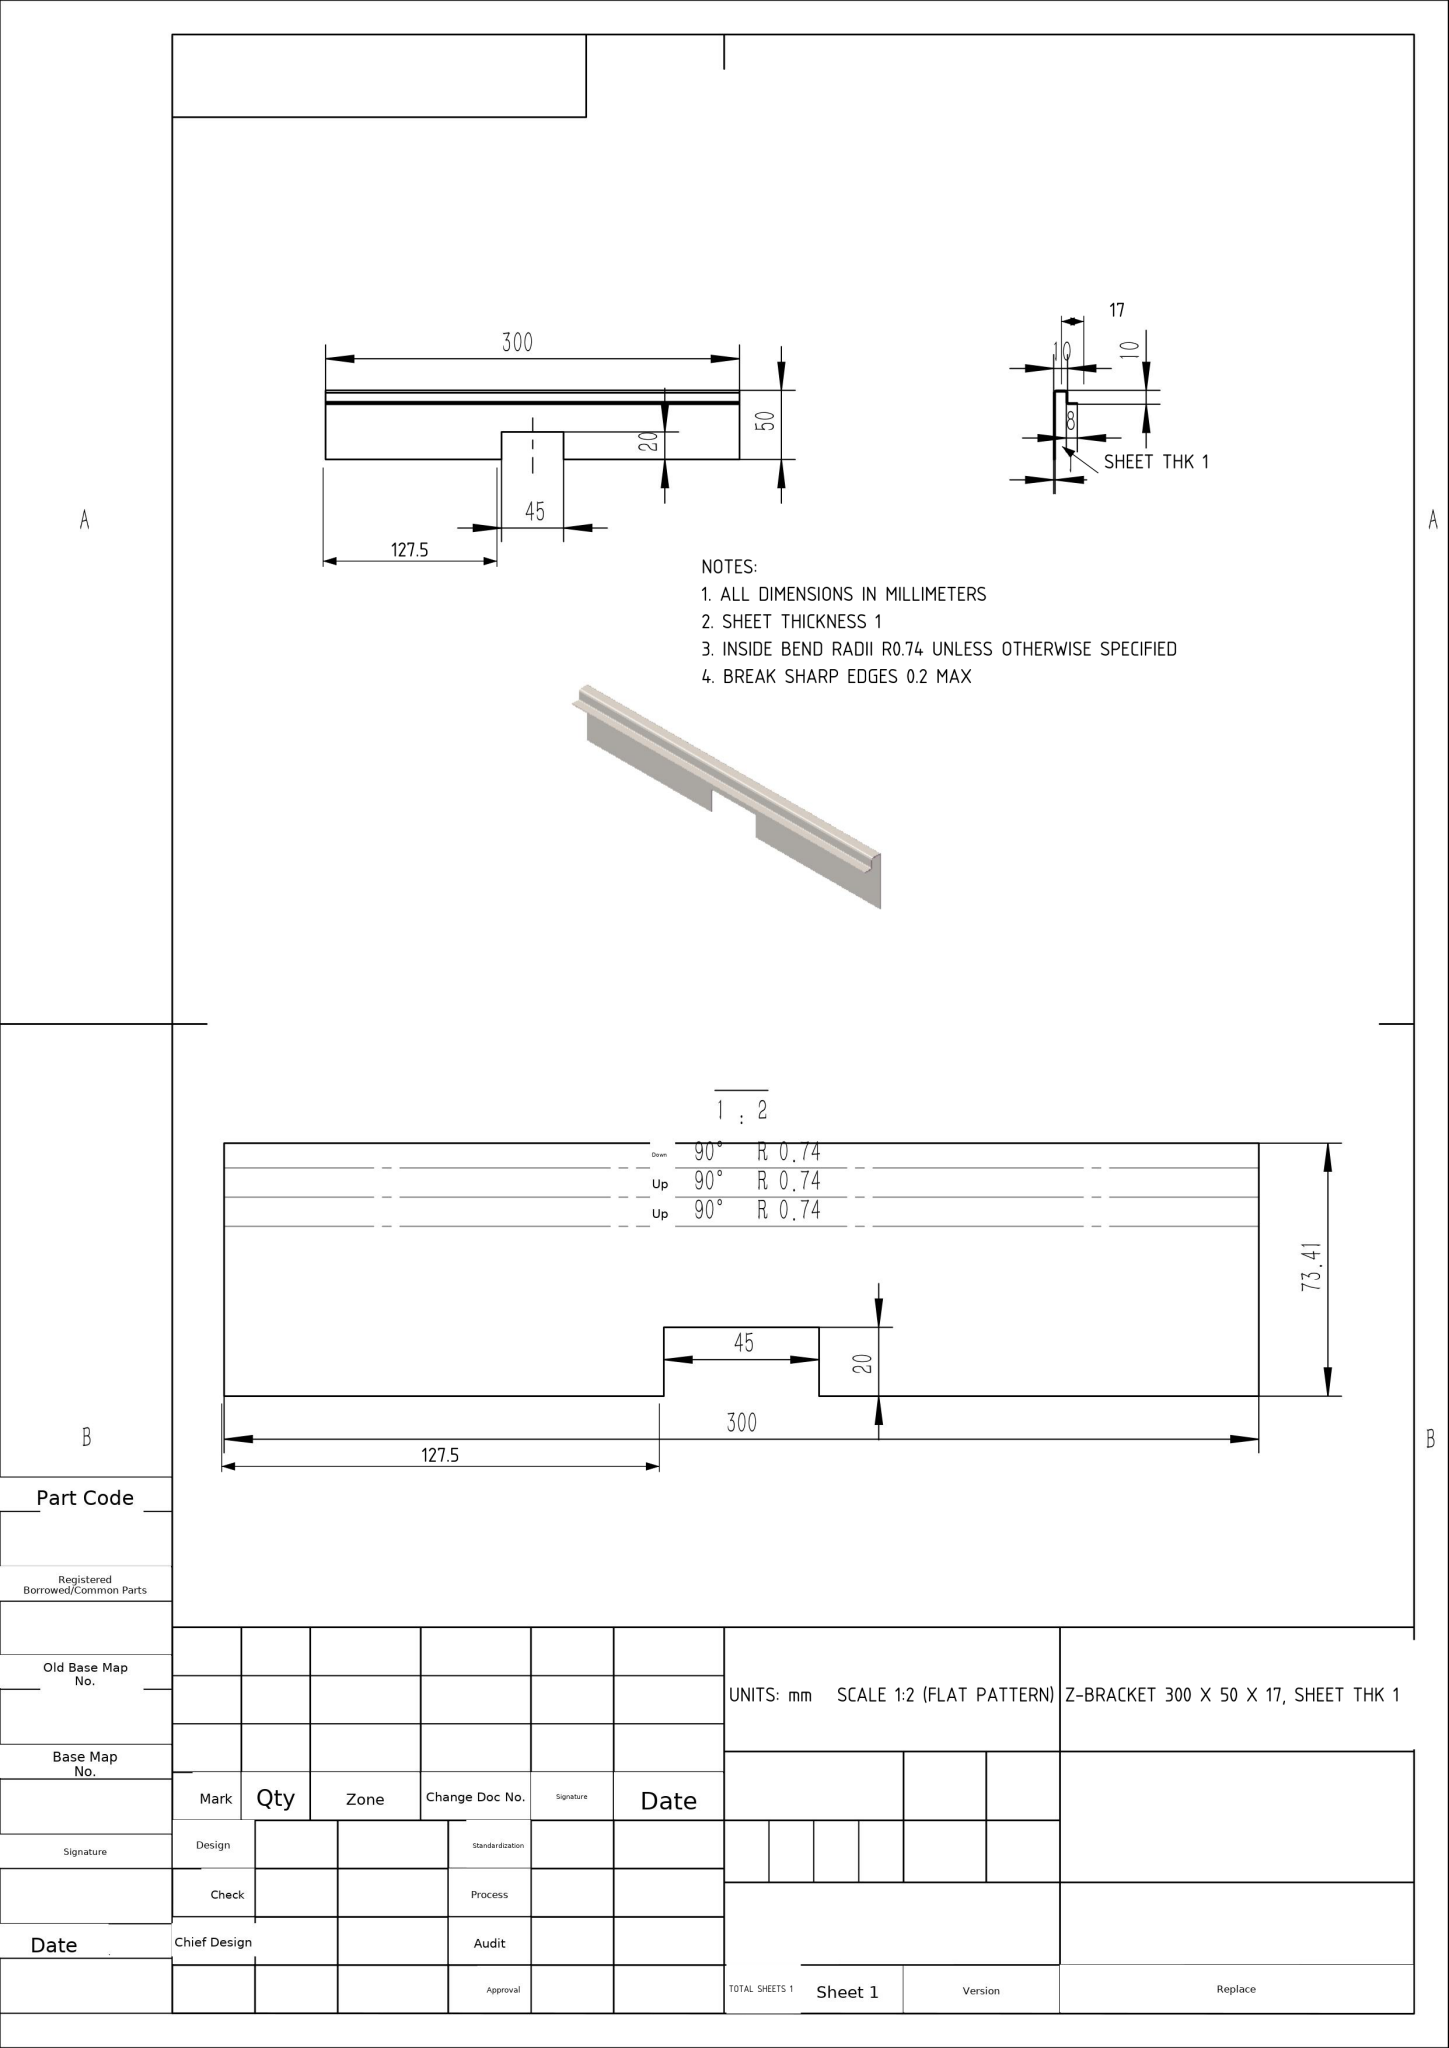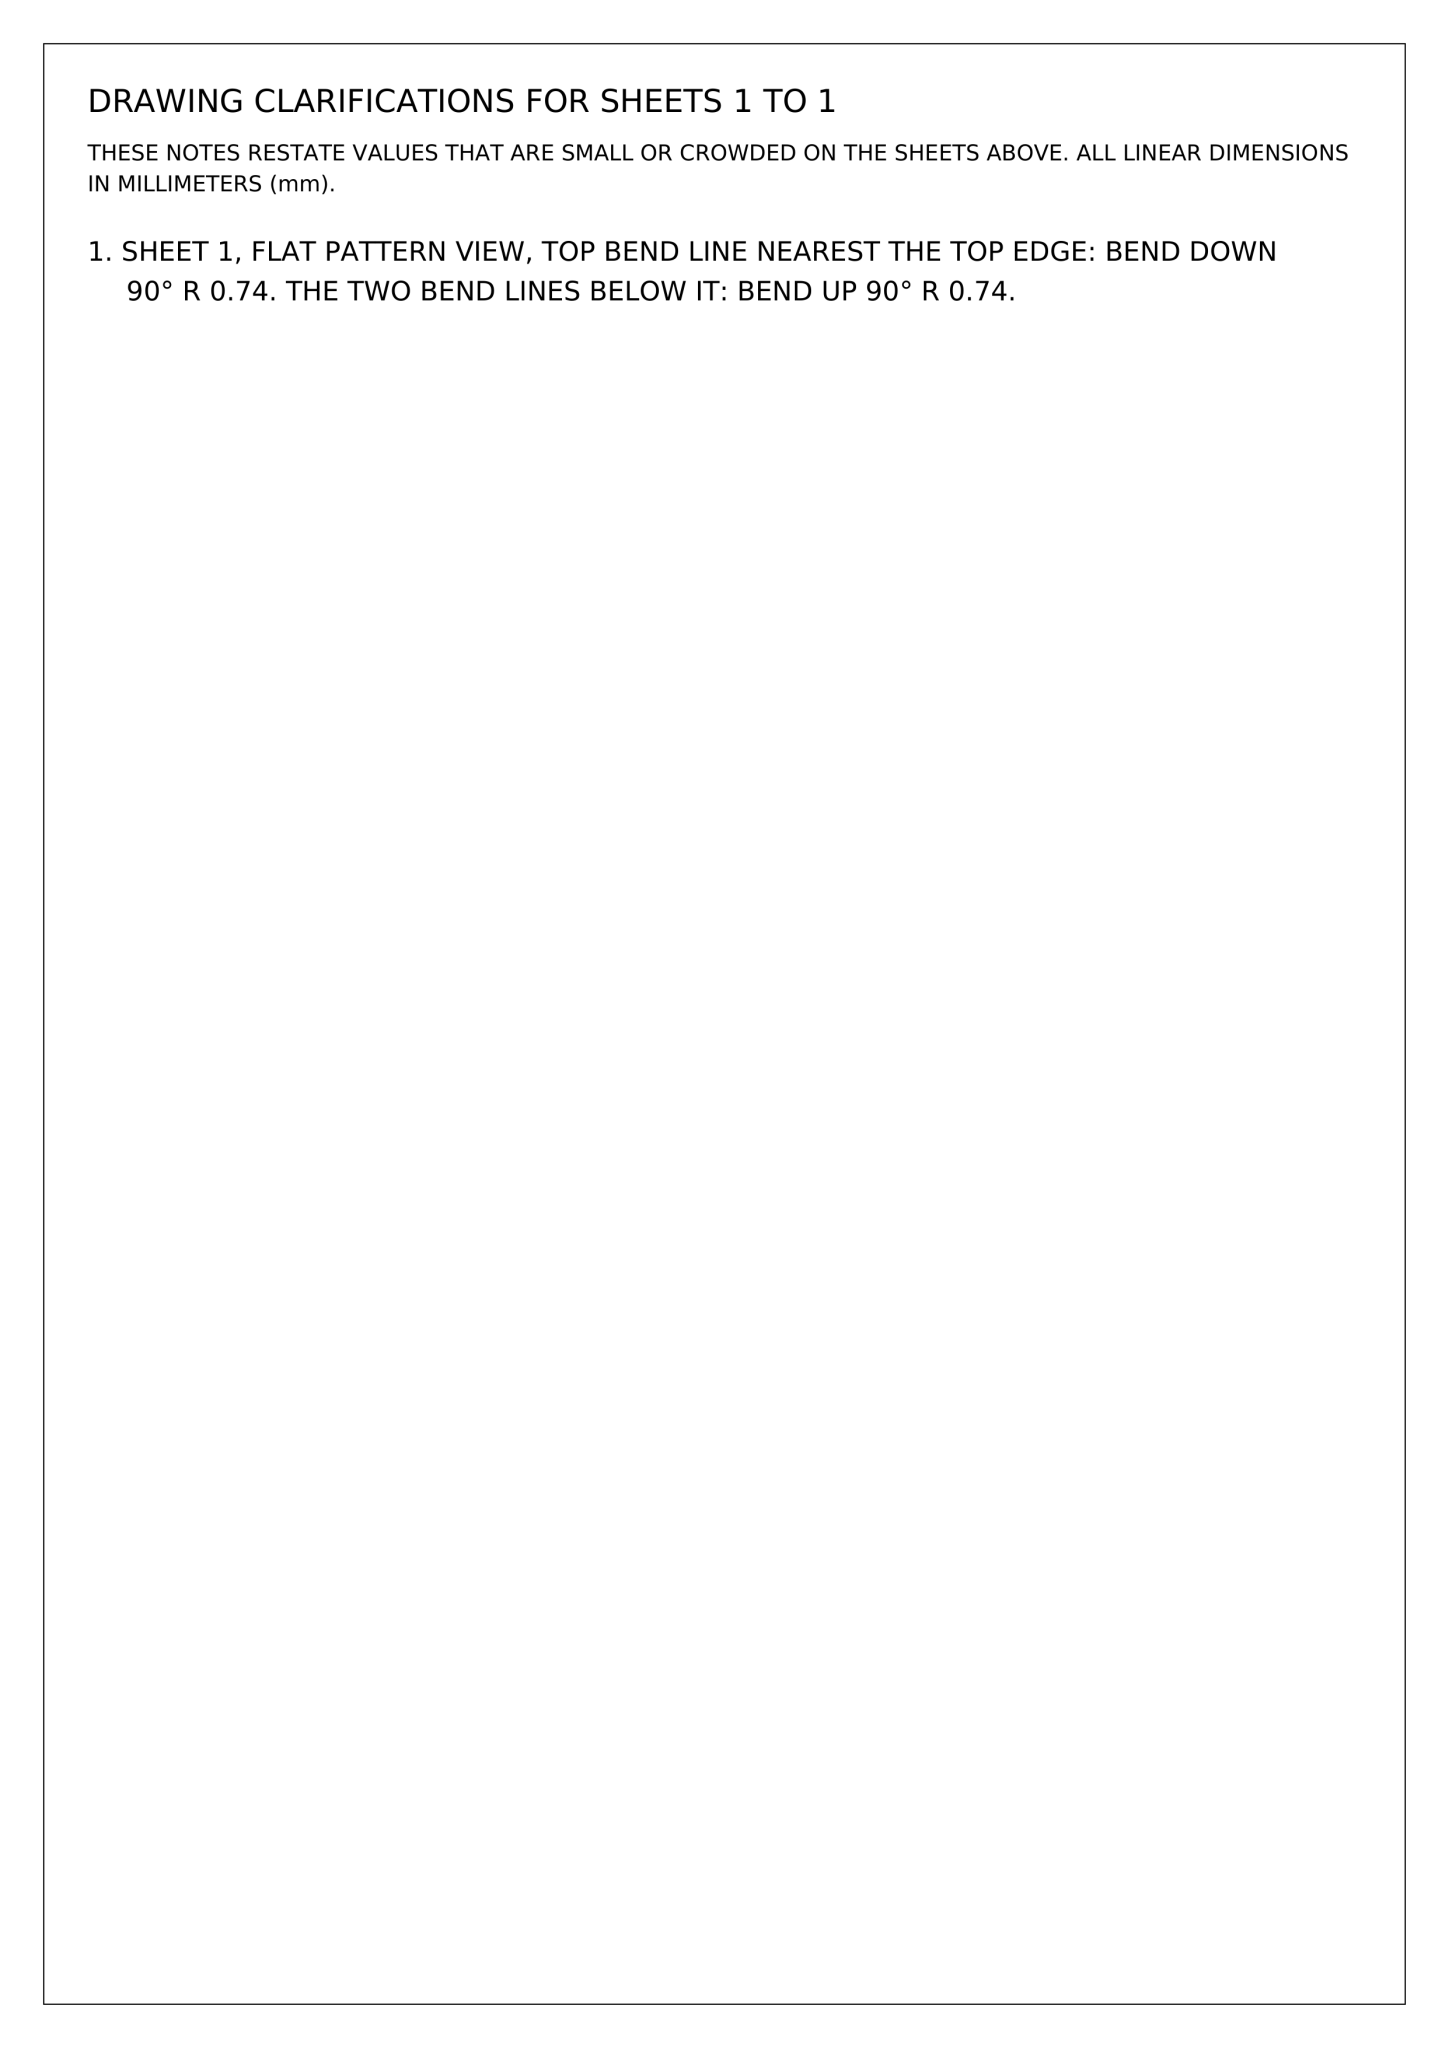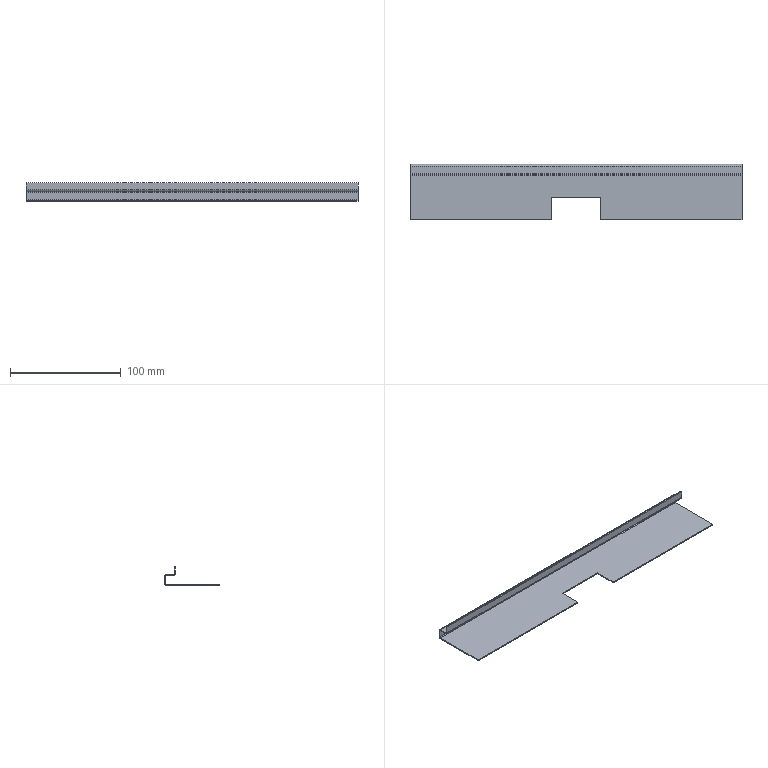Part | NX | mm | 1 solid | 34 faces | box 300 x 50 x 17 mm | volume 21122 mm3 | plane 28 | cylinder 6 | commonest cylinder face diameters 3.473 x3 1.473 x3
STEP:
#1=COLOUR_RGB('',0.6471,0.6196,0.5882);
#2=FILL_AREA_STYLE_COLOUR('',#1);
#3=FILL_AREA_STYLE('',(#2));
#4=SURFACE_STYLE_FILL_AREA(#3);
#5=SURFACE_SIDE_STYLE('',(#4));
#6=SURFACE_STYLE_USAGE(.BOTH.,#5);
#7=PRESENTATION_STYLE_ASSIGNMENT((#6));
#8=CARTESIAN_POINT('',(13.846,64.904,-1.));
#9=VERTEX_POINT('',#8);
#10=CARTESIAN_POINT('',(13.846,64.904,0.));
#11=VERTEX_POINT('',#10);
#12=CARTESIAN_POINT('',(13.846,64.904,-1.));
#13=DIRECTION('',(0.,0.,1.));
#14=VECTOR('',#13,1000.);
#15=LINE('',#12,#14);
#16=EDGE_CURVE('',#9,#11,#15,.T.);
#17=ORIENTED_EDGE('',*,*,#16,.F.);
#18=CARTESIAN_POINT('',(141.346,64.904,-1.));
#19=VERTEX_POINT('',#18);
#20=CARTESIAN_POINT('',(-158.654,64.904,-1.));
#21=DIRECTION('',(1.,0.,0.));
#22=VECTOR('',#21,1000.);
#23=LINE('',#20,#22);
#24=EDGE_CURVE('',#9,#19,#23,.T.);
#25=ORIENTED_EDGE('',*,*,#24,.T.);
#26=CARTESIAN_POINT('',(141.346,64.904,0.));
#27=VERTEX_POINT('',#26);
#28=CARTESIAN_POINT('',(141.346,64.904,-1.));
#29=DIRECTION('',(0.,0.,1.));
#30=VECTOR('',#29,1000.);
#31=LINE('',#28,#30);
#32=EDGE_CURVE('',#19,#27,#31,.T.);
#33=ORIENTED_EDGE('',*,*,#32,.T.);
#34=CARTESIAN_POINT('',(-158.654,64.904,0.));
#35=DIRECTION('',(1.,0.,0.));
#36=VECTOR('',#35,1000.);
#37=LINE('',#34,#36);
#38=EDGE_CURVE('',#11,#27,#37,.T.);
#39=ORIENTED_EDGE('',*,*,#38,.F.);
#40=EDGE_LOOP('',(#17,#25,#33,#39));
#41=FACE_OUTER_BOUND('',#40,.T.);
#42=CARTESIAN_POINT('',(-158.654,64.904,-1.));
#43=DIRECTION('',(0.,-1.,0.));
#44=DIRECTION('',(0.,0.,-1.));
#45=AXIS2_PLACEMENT_3D('',#42,#43,#44);
#46=PLANE('',#45);
#47=ADVANCED_FACE('',(#41),#46,.T.);
#48=CARTESIAN_POINT('',(141.346,113.167,9.));
#49=VERTEX_POINT('',#48);
#50=CARTESIAN_POINT('',(141.346,106.64,9.));
#51=VERTEX_POINT('',#50);
#52=CARTESIAN_POINT('',(141.346,104.904,9.));
#53=DIRECTION('',(0.,-1.,0.));
#54=VECTOR('',#53,1000.);
#55=LINE('',#52,#54);
#56=EDGE_CURVE('',#49,#51,#55,.T.);
#57=ORIENTED_EDGE('',*,*,#56,.T.);
#58=CARTESIAN_POINT('',(141.346,106.64,8.));
#59=VERTEX_POINT('',#58);
#60=CARTESIAN_POINT('',(141.346,106.64,9.));
#61=DIRECTION('',(0.,0.,-1.));
#62=VECTOR('',#61,1000.);
#63=LINE('',#60,#62);
#64=EDGE_CURVE('',#51,#59,#63,.T.);
#65=ORIENTED_EDGE('',*,*,#64,.T.);
#66=CARTESIAN_POINT('',(141.346,113.167,8.));
#67=VERTEX_POINT('',#66);
#68=CARTESIAN_POINT('',(141.346,0.,8.));
#69=DIRECTION('',(0.,-1.,0.));
#70=VECTOR('',#69,1000.);
#71=LINE('',#68,#70);
#72=EDGE_CURVE('',#67,#59,#71,.T.);
#73=ORIENTED_EDGE('',*,*,#72,.F.);
#74=CARTESIAN_POINT('',(141.346,113.167,9.));
#75=DIRECTION('',(0.,0.,1.));
#76=VECTOR('',#75,1000.);
#77=LINE('',#74,#76);
#78=EDGE_CURVE('',#67,#49,#77,.T.);
#79=ORIENTED_EDGE('',*,*,#78,.T.);
#80=EDGE_LOOP('',(#57,#65,#73,#79));
#81=FACE_OUTER_BOUND('',#80,.T.);
#82=CARTESIAN_POINT('',(141.346,104.904,9.));
#83=DIRECTION('',(1.,0.,0.));
#84=DIRECTION('',(0.,0.,-1.));
#85=AXIS2_PLACEMENT_3D('',#82,#83,#84);
#86=PLANE('',#85);
#87=ADVANCED_FACE('',(#81),#86,.T.);
#88=CARTESIAN_POINT('',(-158.654,106.64,9.));
#89=VERTEX_POINT('',#88);
#90=CARTESIAN_POINT('',(-158.654,113.167,9.));
#91=VERTEX_POINT('',#90);
#92=CARTESIAN_POINT('',(-158.654,113.904,9.));
#93=DIRECTION('',(0.,1.,-0.));
#94=VECTOR('',#93,1000.);
#95=LINE('',#92,#94);
#96=EDGE_CURVE('',#89,#91,#95,.T.);
#97=ORIENTED_EDGE('',*,*,#96,.F.);
#98=CARTESIAN_POINT('',(141.346,106.64,9.));
#99=DIRECTION('',(-1.,0.,0.));
#100=VECTOR('',#99,1000.);
#101=LINE('',#98,#100);
#102=EDGE_CURVE('',#51,#89,#101,.T.);
#103=ORIENTED_EDGE('',*,*,#102,.F.);
#104=ORIENTED_EDGE('',*,*,#56,.F.);
#105=CARTESIAN_POINT('',(0.,113.167,9.));
#106=DIRECTION('',(-1.,0.,0.));
#107=VECTOR('',#106,1000.);
#108=LINE('',#105,#107);
#109=EDGE_CURVE('',#49,#91,#108,.T.);
#110=ORIENTED_EDGE('',*,*,#109,.T.);
#111=EDGE_LOOP('',(#97,#103,#104,#110));
#112=FACE_OUTER_BOUND('',#111,.T.);
#113=CARTESIAN_POINT('',(0.,0.,9.));
#114=DIRECTION('',(0.,0.,1.));
#115=DIRECTION('',(0.,-1.,0.));
#116=AXIS2_PLACEMENT_3D('',#113,#114,#115);
#117=PLANE('',#116);
#118=ADVANCED_FACE('',(#112),#117,.T.);
#119=CARTESIAN_POINT('',(-158.654,106.64,8.));
#120=VERTEX_POINT('',#119);
#121=CARTESIAN_POINT('',(141.346,106.64,8.));
#122=DIRECTION('',(-1.,0.,0.));
#123=VECTOR('',#122,1000.);
#124=LINE('',#121,#123);
#125=EDGE_CURVE('',#59,#120,#124,.T.);
#126=ORIENTED_EDGE('',*,*,#125,.T.);
#127=CARTESIAN_POINT('',(-158.654,113.167,8.));
#128=VERTEX_POINT('',#127);
#129=CARTESIAN_POINT('',(-158.654,0.,8.));
#130=DIRECTION('',(0.,1.,-0.));
#131=VECTOR('',#130,1000.);
#132=LINE('',#129,#131);
#133=EDGE_CURVE('',#120,#128,#132,.T.);
#134=ORIENTED_EDGE('',*,*,#133,.T.);
#135=CARTESIAN_POINT('',(141.346,113.167,8.));
#136=DIRECTION('',(-1.,0.,0.));
#137=VECTOR('',#136,1000.);
#138=LINE('',#135,#137);
#139=EDGE_CURVE('',#67,#128,#138,.T.);
#140=ORIENTED_EDGE('',*,*,#139,.F.);
#141=ORIENTED_EDGE('',*,*,#72,.T.);
#142=EDGE_LOOP('',(#126,#134,#140,#141));
#143=FACE_OUTER_BOUND('',#142,.T.);
#144=CARTESIAN_POINT('',(0.,0.,8.));
#145=DIRECTION('',(0.,0.,1.));
#146=DIRECTION('',(0.,-1.,0.));
#147=AXIS2_PLACEMENT_3D('',#144,#145,#146);
#148=PLANE('',#147);
#149=ADVANCED_FACE('',(#143),#148,.F.);
#150=CARTESIAN_POINT('',(141.346,113.904,7.263));
#151=VERTEX_POINT('',#150);
#152=CARTESIAN_POINT('',(141.346,114.904,7.263));
#153=VERTEX_POINT('',#152);
#154=CARTESIAN_POINT('',(141.346,113.904,7.263));
#155=DIRECTION('',(0.,1.,-0.));
#156=VECTOR('',#155,1000.);
#157=LINE('',#154,#156);
#158=EDGE_CURVE('',#151,#153,#157,.T.);
#159=ORIENTED_EDGE('',*,*,#158,.F.);
#160=CARTESIAN_POINT('',(141.346,113.904,0.7366));
#161=VERTEX_POINT('',#160);
#162=CARTESIAN_POINT('',(141.346,113.904,-0.));
#163=DIRECTION('',(0.,-0.,-1.));
#164=VECTOR('',#163,1000.);
#165=LINE('',#162,#164);
#166=EDGE_CURVE('',#151,#161,#165,.T.);
#167=ORIENTED_EDGE('',*,*,#166,.T.);
#168=CARTESIAN_POINT('',(141.346,114.904,0.7366));
#169=VERTEX_POINT('',#168);
#170=CARTESIAN_POINT('',(141.346,114.904,0.7366));
#171=DIRECTION('',(0.,1.,-0.));
#172=VECTOR('',#171,1000.);
#173=LINE('',#170,#172);
#174=EDGE_CURVE('',#161,#169,#173,.T.);
#175=ORIENTED_EDGE('',*,*,#174,.T.);
#176=CARTESIAN_POINT('',(141.346,114.904,-0.));
#177=DIRECTION('',(0.,-0.,-1.));
#178=VECTOR('',#177,1000.);
#179=LINE('',#176,#178);
#180=EDGE_CURVE('',#153,#169,#179,.T.);
#181=ORIENTED_EDGE('',*,*,#180,.F.);
#182=EDGE_LOOP('',(#159,#167,#175,#181));
#183=FACE_OUTER_BOUND('',#182,.T.);
#184=CARTESIAN_POINT('',(141.346,114.904,-0.));
#185=DIRECTION('',(-1.,0.,0.));
#186=DIRECTION('',(0.,0.,1.));
#187=AXIS2_PLACEMENT_3D('',#184,#185,#186);
#188=PLANE('',#187);
#189=ADVANCED_FACE('',(#183),#188,.F.);
#190=CARTESIAN_POINT('',(-158.654,113.904,7.263));
#191=VERTEX_POINT('',#190);
#192=CARTESIAN_POINT('',(-158.654,114.904,7.263));
#193=VERTEX_POINT('',#192);
#194=CARTESIAN_POINT('',(-158.654,113.904,7.263));
#195=DIRECTION('',(0.,1.,-0.));
#196=VECTOR('',#195,1000.);
#197=LINE('',#194,#196);
#198=EDGE_CURVE('',#191,#193,#197,.T.);
#199=ORIENTED_EDGE('',*,*,#198,.T.);
#200=CARTESIAN_POINT('',(-158.654,114.904,0.7366));
#201=VERTEX_POINT('',#200);
#202=CARTESIAN_POINT('',(-158.654,114.904,-0.));
#203=DIRECTION('',(0.,0.,1.));
#204=VECTOR('',#203,1000.);
#205=LINE('',#202,#204);
#206=EDGE_CURVE('',#201,#193,#205,.T.);
#207=ORIENTED_EDGE('',*,*,#206,.F.);
#208=CARTESIAN_POINT('',(-158.654,113.904,0.7366));
#209=VERTEX_POINT('',#208);
#210=CARTESIAN_POINT('',(-158.654,113.904,0.7366));
#211=DIRECTION('',(0.,1.,-0.));
#212=VECTOR('',#211,1000.);
#213=LINE('',#210,#212);
#214=EDGE_CURVE('',#209,#201,#213,.T.);
#215=ORIENTED_EDGE('',*,*,#214,.F.);
#216=CARTESIAN_POINT('',(-158.654,113.904,9.));
#217=DIRECTION('',(0.,0.,1.));
#218=VECTOR('',#217,1000.);
#219=LINE('',#216,#218);
#220=EDGE_CURVE('',#209,#191,#219,.T.);
#221=ORIENTED_EDGE('',*,*,#220,.T.);
#222=EDGE_LOOP('',(#199,#207,#215,#221));
#223=FACE_OUTER_BOUND('',#222,.T.);
#224=CARTESIAN_POINT('',(-158.654,114.904,9.));
#225=DIRECTION('',(1.,0.,0.));
#226=DIRECTION('',(0.,0.,-1.));
#227=AXIS2_PLACEMENT_3D('',#224,#225,#226);
#228=PLANE('',#227);
#229=ADVANCED_FACE('',(#223),#228,.F.);
#230=CARTESIAN_POINT('',(-158.654,114.904,7.263));
#231=DIRECTION('',(1.,0.,0.));
#232=VECTOR('',#231,1000.);
#233=LINE('',#230,#232);
#234=EDGE_CURVE('',#193,#153,#233,.T.);
#235=ORIENTED_EDGE('',*,*,#234,.T.);
#236=ORIENTED_EDGE('',*,*,#180,.T.);
#237=CARTESIAN_POINT('',(141.346,114.904,0.7366));
#238=DIRECTION('',(1.,-0.,-0.));
#239=VECTOR('',#238,1000.);
#240=LINE('',#237,#239);
#241=EDGE_CURVE('',#201,#169,#240,.T.);
#242=ORIENTED_EDGE('',*,*,#241,.F.);
#243=ORIENTED_EDGE('',*,*,#206,.T.);
#244=EDGE_LOOP('',(#235,#236,#242,#243));
#245=FACE_OUTER_BOUND('',#244,.T.);
#246=CARTESIAN_POINT('',(0.,114.904,-0.));
#247=DIRECTION('',(0.,-1.,0.));
#248=DIRECTION('',(0.,-0.,-1.));
#249=AXIS2_PLACEMENT_3D('',#246,#247,#248);
#250=PLANE('',#249);
#251=ADVANCED_FACE('',(#245),#250,.F.);
#252=ORIENTED_EDGE('',*,*,#166,.F.);
#253=CARTESIAN_POINT('',(-158.654,113.904,7.263));
#254=DIRECTION('',(1.,0.,0.));
#255=VECTOR('',#254,1000.);
#256=LINE('',#253,#255);
#257=EDGE_CURVE('',#191,#151,#256,.T.);
#258=ORIENTED_EDGE('',*,*,#257,.F.);
#259=ORIENTED_EDGE('',*,*,#220,.F.);
#260=CARTESIAN_POINT('',(141.346,113.904,0.7366));
#261=DIRECTION('',(-1.,0.,0.));
#262=VECTOR('',#261,1000.);
#263=LINE('',#260,#262);
#264=EDGE_CURVE('',#161,#209,#263,.T.);
#265=ORIENTED_EDGE('',*,*,#264,.F.);
#266=EDGE_LOOP('',(#252,#258,#259,#265));
#267=FACE_OUTER_BOUND('',#266,.T.);
#268=CARTESIAN_POINT('',(0.,113.904,-0.));
#269=DIRECTION('',(0.,-1.,0.));
#270=DIRECTION('',(0.,-0.,-1.));
#271=AXIS2_PLACEMENT_3D('',#268,#269,#270);
#272=PLANE('',#271);
#273=ADVANCED_FACE('',(#267),#272,.T.);
#274=CARTESIAN_POINT('',(-158.654,113.167,0.));
#275=VERTEX_POINT('',#274);
#276=CARTESIAN_POINT('',(-158.654,64.904,0.));
#277=VERTEX_POINT('',#276);
#278=CARTESIAN_POINT('',(-158.654,114.904,0.));
#279=DIRECTION('',(-0.,-1.,0.));
#280=VECTOR('',#279,1000.);
#281=LINE('',#278,#280);
#282=EDGE_CURVE('',#275,#277,#281,.T.);
#283=ORIENTED_EDGE('',*,*,#282,.F.);
#284=CARTESIAN_POINT('',(-158.654,113.167,-1.));
#285=VERTEX_POINT('',#284);
#286=CARTESIAN_POINT('',(-158.654,113.167,0.));
#287=DIRECTION('',(-0.,0.,-1.));
#288=VECTOR('',#287,1000.);
#289=LINE('',#286,#288);
#290=EDGE_CURVE('',#275,#285,#289,.T.);
#291=ORIENTED_EDGE('',*,*,#290,.T.);
#292=CARTESIAN_POINT('',(-158.654,64.904,-1.));
#293=VERTEX_POINT('',#292);
#294=CARTESIAN_POINT('',(-158.654,114.904,-1.));
#295=DIRECTION('',(-0.,-1.,0.));
#296=VECTOR('',#295,1000.);
#297=LINE('',#294,#296);
#298=EDGE_CURVE('',#285,#293,#297,.T.);
#299=ORIENTED_EDGE('',*,*,#298,.T.);
#300=CARTESIAN_POINT('',(-158.654,64.904,-1.));
#301=DIRECTION('',(0.,0.,1.));
#302=VECTOR('',#301,1000.);
#303=LINE('',#300,#302);
#304=EDGE_CURVE('',#293,#277,#303,.T.);
#305=ORIENTED_EDGE('',*,*,#304,.T.);
#306=EDGE_LOOP('',(#283,#291,#299,#305));
#307=FACE_OUTER_BOUND('',#306,.T.);
#308=CARTESIAN_POINT('',(-158.654,114.904,-1.));
#309=DIRECTION('',(-1.,0.,0.));
#310=DIRECTION('',(-0.,-1.,0.));
#311=AXIS2_PLACEMENT_3D('',#308,#309,#310);
#312=PLANE('',#311);
#313=ADVANCED_FACE('',(#307),#312,.T.);
#314=ORIENTED_EDGE('',*,*,#24,.F.);
#315=CARTESIAN_POINT('',(13.846,84.904,-1.));
#316=VERTEX_POINT('',#315);
#317=CARTESIAN_POINT('',(13.846,0.,-1.));
#318=DIRECTION('',(0.,1.,0.));
#319=VECTOR('',#318,1000.);
#320=LINE('',#317,#319);
#321=EDGE_CURVE('',#9,#316,#320,.T.);
#322=ORIENTED_EDGE('',*,*,#321,.T.);
#323=CARTESIAN_POINT('',(-31.154,84.904,-1.));
#324=VERTEX_POINT('',#323);
#325=CARTESIAN_POINT('',(0.,84.904,-1.));
#326=DIRECTION('',(-1.,0.,0.));
#327=VECTOR('',#326,1000.);
#328=LINE('',#325,#327);
#329=EDGE_CURVE('',#316,#324,#328,.T.);
#330=ORIENTED_EDGE('',*,*,#329,.T.);
#331=CARTESIAN_POINT('',(-31.154,64.904,-1.));
#332=VERTEX_POINT('',#331);
#333=CARTESIAN_POINT('',(-31.154,0.,-1.));
#334=DIRECTION('',(-0.,-1.,0.));
#335=VECTOR('',#334,1000.);
#336=LINE('',#333,#335);
#337=EDGE_CURVE('',#324,#332,#336,.T.);
#338=ORIENTED_EDGE('',*,*,#337,.T.);
#339=CARTESIAN_POINT('',(-158.654,64.904,-1.));
#340=DIRECTION('',(1.,0.,0.));
#341=VECTOR('',#340,1000.);
#342=LINE('',#339,#341);
#343=EDGE_CURVE('',#293,#332,#342,.T.);
#344=ORIENTED_EDGE('',*,*,#343,.F.);
#345=ORIENTED_EDGE('',*,*,#298,.F.);
#346=CARTESIAN_POINT('',(141.346,113.167,-1.));
#347=VERTEX_POINT('',#346);
#348=CARTESIAN_POINT('',(-158.654,113.167,-1.));
#349=DIRECTION('',(1.,0.,-0.));
#350=VECTOR('',#349,1000.);
#351=LINE('',#348,#350);
#352=EDGE_CURVE('',#285,#347,#351,.T.);
#353=ORIENTED_EDGE('',*,*,#352,.T.);
#354=CARTESIAN_POINT('',(141.346,64.904,-1.));
#355=DIRECTION('',(0.,1.,0.));
#356=VECTOR('',#355,1000.);
#357=LINE('',#354,#356);
#358=EDGE_CURVE('',#19,#347,#357,.T.);
#359=ORIENTED_EDGE('',*,*,#358,.F.);
#360=EDGE_LOOP('',(#314,#322,#330,#338,#344,#345,#353,#359));
#361=FACE_OUTER_BOUND('',#360,.T.);
#362=CARTESIAN_POINT('',(0.,0.,-1.));
#363=DIRECTION('',(0.,0.,1.));
#364=DIRECTION('',(1.,0.,0.));
#365=AXIS2_PLACEMENT_3D('',#362,#363,#364);
#366=PLANE('',#365);
#367=ADVANCED_FACE('',(#361),#366,.F.);
#368=CARTESIAN_POINT('',(13.846,84.904,0.));
#369=VERTEX_POINT('',#368);
#370=CARTESIAN_POINT('',(13.846,0.,0.));
#371=DIRECTION('',(0.,1.,0.));
#372=VECTOR('',#371,1000.);
#373=LINE('',#370,#372);
#374=EDGE_CURVE('',#11,#369,#373,.T.);
#375=ORIENTED_EDGE('',*,*,#374,.F.);
#376=ORIENTED_EDGE('',*,*,#38,.T.);
#377=CARTESIAN_POINT('',(141.346,113.167,-0.));
#378=VERTEX_POINT('',#377);
#379=CARTESIAN_POINT('',(141.346,64.904,0.));
#380=DIRECTION('',(0.,1.,0.));
#381=VECTOR('',#380,1000.);
#382=LINE('',#379,#381);
#383=EDGE_CURVE('',#27,#378,#382,.T.);
#384=ORIENTED_EDGE('',*,*,#383,.T.);
#385=CARTESIAN_POINT('',(-158.654,113.167,0.));
#386=DIRECTION('',(1.,0.,-0.));
#387=VECTOR('',#386,1000.);
#388=LINE('',#385,#387);
#389=EDGE_CURVE('',#275,#378,#388,.T.);
#390=ORIENTED_EDGE('',*,*,#389,.F.);
#391=ORIENTED_EDGE('',*,*,#282,.T.);
#392=CARTESIAN_POINT('',(-31.154,64.904,0.));
#393=VERTEX_POINT('',#392);
#394=CARTESIAN_POINT('',(-158.654,64.904,0.));
#395=DIRECTION('',(1.,0.,0.));
#396=VECTOR('',#395,1000.);
#397=LINE('',#394,#396);
#398=EDGE_CURVE('',#277,#393,#397,.T.);
#399=ORIENTED_EDGE('',*,*,#398,.T.);
#400=CARTESIAN_POINT('',(-31.154,84.904,0.));
#401=VERTEX_POINT('',#400);
#402=CARTESIAN_POINT('',(-31.154,0.,0.));
#403=DIRECTION('',(-0.,-1.,0.));
#404=VECTOR('',#403,1000.);
#405=LINE('',#402,#404);
#406=EDGE_CURVE('',#401,#393,#405,.T.);
#407=ORIENTED_EDGE('',*,*,#406,.F.);
#408=CARTESIAN_POINT('',(0.,84.904,0.));
#409=DIRECTION('',(-1.,0.,0.));
#410=VECTOR('',#409,1000.);
#411=LINE('',#408,#410);
#412=EDGE_CURVE('',#369,#401,#411,.T.);
#413=ORIENTED_EDGE('',*,*,#412,.F.);
#414=EDGE_LOOP('',(#375,#376,#384,#390,#391,#399,#407,#413));
#415=FACE_OUTER_BOUND('',#414,.T.);
#416=CARTESIAN_POINT('',(0.,0.,0.));
#417=DIRECTION('',(0.,0.,1.));
#418=DIRECTION('',(1.,0.,0.));
#419=AXIS2_PLACEMENT_3D('',#416,#417,#418);
#420=PLANE('',#419);
#421=ADVANCED_FACE('',(#415),#420,.T.);
#422=CARTESIAN_POINT('',(141.346,113.167,-0.));
#423=DIRECTION('',(0.,0.,-1.));
#424=VECTOR('',#423,1000.);
#425=LINE('',#422,#424);
#426=EDGE_CURVE('',#378,#347,#425,.T.);
#427=ORIENTED_EDGE('',*,*,#426,.F.);
#428=ORIENTED_EDGE('',*,*,#383,.F.);
#429=ORIENTED_EDGE('',*,*,#32,.F.);
#430=ORIENTED_EDGE('',*,*,#358,.T.);
#431=EDGE_LOOP('',(#427,#428,#429,#430));
#432=FACE_OUTER_BOUND('',#431,.T.);
#433=CARTESIAN_POINT('',(141.346,64.904,-1.));
#434=DIRECTION('',(1.,-0.,0.));
#435=DIRECTION('',(0.,1.,0.));
#436=AXIS2_PLACEMENT_3D('',#433,#434,#435);
#437=PLANE('',#436);
#438=ADVANCED_FACE('',(#432),#437,.T.);
#439=CARTESIAN_POINT('',(-31.154,64.904,-1.));
#440=DIRECTION('',(0.,0.,-1.));
#441=VECTOR('',#440,1000.);
#442=LINE('',#439,#441);
#443=EDGE_CURVE('',#393,#332,#442,.T.);
#444=ORIENTED_EDGE('',*,*,#443,.F.);
#445=ORIENTED_EDGE('',*,*,#398,.F.);
#446=ORIENTED_EDGE('',*,*,#304,.F.);
#447=ORIENTED_EDGE('',*,*,#343,.T.);
#448=EDGE_LOOP('',(#444,#445,#446,#447));
#449=FACE_OUTER_BOUND('',#448,.T.);
#450=CARTESIAN_POINT('',(-158.654,64.904,-1.));
#451=DIRECTION('',(0.,-1.,0.));
#452=DIRECTION('',(0.,0.,-1.));
#453=AXIS2_PLACEMENT_3D('',#450,#451,#452);
#454=PLANE('',#453);
#455=ADVANCED_FACE('',(#449),#454,.T.);
#456=ORIENTED_EDGE('',*,*,#174,.F.);
#457=CARTESIAN_POINT('',(141.346,113.167,0.7366));
#458=DIRECTION('',(1.,0.,-0.));
#459=DIRECTION('',(0.,0.,1.));
#460=AXIS2_PLACEMENT_3D('',#457,#458,#459);
#461=CIRCLE('',#460,0.7366);
#462=EDGE_CURVE('',#378,#161,#461,.T.);
#463=ORIENTED_EDGE('',*,*,#462,.F.);
#464=ORIENTED_EDGE('',*,*,#426,.T.);
#465=CARTESIAN_POINT('',(141.346,113.167,0.7366));
#466=DIRECTION('',(1.,0.,-0.));
#467=DIRECTION('',(0.,0.,1.));
#468=AXIS2_PLACEMENT_3D('',#465,#466,#467);
#469=CIRCLE('',#468,1.737);
#470=EDGE_CURVE('',#347,#169,#469,.T.);
#471=ORIENTED_EDGE('',*,*,#470,.T.);
#472=EDGE_LOOP('',(#456,#463,#464,#471));
#473=FACE_OUTER_BOUND('',#472,.T.);
#474=CARTESIAN_POINT('',(141.346,113.167,0.7366));
#475=DIRECTION('',(1.,0.,-0.));
#476=DIRECTION('',(-0.,0.,-1.));
#477=AXIS2_PLACEMENT_3D('',#474,#475,#476);
#478=PLANE('',#477);
#479=ADVANCED_FACE('',(#473),#478,.T.);
#480=CARTESIAN_POINT('',(-158.654,113.167,0.7366));
#481=DIRECTION('',(-1.,0.,0.));
#482=DIRECTION('',(0.,0.,1.));
#483=AXIS2_PLACEMENT_3D('',#480,#481,#482);
#484=CIRCLE('',#483,0.7366);
#485=EDGE_CURVE('',#209,#275,#484,.T.);
#486=ORIENTED_EDGE('',*,*,#485,.F.);
#487=ORIENTED_EDGE('',*,*,#214,.T.);
#488=CARTESIAN_POINT('',(-158.654,113.167,0.7366));
#489=DIRECTION('',(-1.,0.,0.));
#490=DIRECTION('',(0.,0.,1.));
#491=AXIS2_PLACEMENT_3D('',#488,#489,#490);
#492=CIRCLE('',#491,1.737);
#493=EDGE_CURVE('',#201,#285,#492,.T.);
#494=ORIENTED_EDGE('',*,*,#493,.T.);
#495=ORIENTED_EDGE('',*,*,#290,.F.);
#496=EDGE_LOOP('',(#486,#487,#494,#495));
#497=FACE_OUTER_BOUND('',#496,.T.);
#498=CARTESIAN_POINT('',(-158.654,113.167,0.7366));
#499=DIRECTION('',(1.,0.,-0.));
#500=DIRECTION('',(-0.,0.,-1.));
#501=AXIS2_PLACEMENT_3D('',#498,#499,#500);
#502=PLANE('',#501);
#503=ADVANCED_FACE('',(#497),#502,.F.);
#504=ORIENTED_EDGE('',*,*,#352,.F.);
#505=ORIENTED_EDGE('',*,*,#493,.F.);
#506=ORIENTED_EDGE('',*,*,#241,.T.);
#507=ORIENTED_EDGE('',*,*,#470,.F.);
#508=EDGE_LOOP('',(#504,#505,#506,#507));
#509=FACE_OUTER_BOUND('',#508,.T.);
#510=CARTESIAN_POINT('',(-158.654,113.167,0.7366));
#511=DIRECTION('',(-1.,0.,0.));
#512=DIRECTION('',(0.,1.,-0.));
#513=AXIS2_PLACEMENT_3D('',#510,#511,#512);
#514=CYLINDRICAL_SURFACE('',#513,1.737);
#515=ADVANCED_FACE('',(#509),#514,.T.);
#516=ORIENTED_EDGE('',*,*,#389,.T.);
#517=ORIENTED_EDGE('',*,*,#462,.T.);
#518=ORIENTED_EDGE('',*,*,#264,.T.);
#519=ORIENTED_EDGE('',*,*,#485,.T.);
#520=EDGE_LOOP('',(#516,#517,#518,#519));
#521=FACE_OUTER_BOUND('',#520,.T.);
#522=CARTESIAN_POINT('',(-158.654,113.167,0.7366));
#523=DIRECTION('',(-1.,0.,0.));
#524=DIRECTION('',(0.,1.,-0.));
#525=AXIS2_PLACEMENT_3D('',#522,#523,#524);
#526=CYLINDRICAL_SURFACE('',#525,0.7366);
#527=ADVANCED_FACE('',(#521),#526,.F.);
#528=ORIENTED_EDGE('',*,*,#78,.F.);
#529=CARTESIAN_POINT('',(141.346,113.167,7.263));
#530=DIRECTION('',(1.,0.,0.));
#531=DIRECTION('',(0.,0.,1.));
#532=AXIS2_PLACEMENT_3D('',#529,#530,#531);
#533=CIRCLE('',#532,0.7366);
#534=EDGE_CURVE('',#151,#67,#533,.T.);
#535=ORIENTED_EDGE('',*,*,#534,.F.);
#536=ORIENTED_EDGE('',*,*,#158,.T.);
#537=CARTESIAN_POINT('',(141.346,113.167,7.263));
#538=DIRECTION('',(1.,0.,0.));
#539=DIRECTION('',(0.,0.,1.));
#540=AXIS2_PLACEMENT_3D('',#537,#538,#539);
#541=CIRCLE('',#540,1.737);
#542=EDGE_CURVE('',#153,#49,#541,.T.);
#543=ORIENTED_EDGE('',*,*,#542,.T.);
#544=EDGE_LOOP('',(#528,#535,#536,#543));
#545=FACE_OUTER_BOUND('',#544,.T.);
#546=CARTESIAN_POINT('',(141.346,113.167,7.263));
#547=DIRECTION('',(1.,0.,0.));
#548=DIRECTION('',(0.,0.,-1.));
#549=AXIS2_PLACEMENT_3D('',#546,#547,#548);
#550=PLANE('',#549);
#551=ADVANCED_FACE('',(#545),#550,.T.);
#552=CARTESIAN_POINT('',(-158.654,113.167,7.263));
#553=DIRECTION('',(-1.,0.,0.));
#554=DIRECTION('',(0.,0.,1.));
#555=AXIS2_PLACEMENT_3D('',#552,#553,#554);
#556=CIRCLE('',#555,0.7366);
#557=EDGE_CURVE('',#128,#191,#556,.T.);
#558=ORIENTED_EDGE('',*,*,#557,.F.);
#559=CARTESIAN_POINT('',(-158.654,113.167,8.));
#560=DIRECTION('',(0.,0.,1.));
#561=VECTOR('',#560,1000.);
#562=LINE('',#559,#561);
#563=EDGE_CURVE('',#128,#91,#562,.T.);
#564=ORIENTED_EDGE('',*,*,#563,.T.);
#565=CARTESIAN_POINT('',(-158.654,113.167,7.263));
#566=DIRECTION('',(-1.,0.,0.));
#567=DIRECTION('',(0.,0.,1.));
#568=AXIS2_PLACEMENT_3D('',#565,#566,#567);
#569=CIRCLE('',#568,1.737);
#570=EDGE_CURVE('',#91,#193,#569,.T.);
#571=ORIENTED_EDGE('',*,*,#570,.T.);
#572=ORIENTED_EDGE('',*,*,#198,.F.);
#573=EDGE_LOOP('',(#558,#564,#571,#572));
#574=FACE_OUTER_BOUND('',#573,.T.);
#575=CARTESIAN_POINT('',(-158.654,113.167,7.263));
#576=DIRECTION('',(1.,0.,0.));
#577=DIRECTION('',(0.,0.,-1.));
#578=AXIS2_PLACEMENT_3D('',#575,#576,#577);
#579=PLANE('',#578);
#580=ADVANCED_FACE('',(#574),#579,.F.);
#581=ORIENTED_EDGE('',*,*,#234,.F.);
#582=ORIENTED_EDGE('',*,*,#570,.F.);
#583=ORIENTED_EDGE('',*,*,#109,.F.);
#584=ORIENTED_EDGE('',*,*,#542,.F.);
#585=EDGE_LOOP('',(#581,#582,#583,#584));
#586=FACE_OUTER_BOUND('',#585,.T.);
#587=CARTESIAN_POINT('',(-158.654,113.167,7.263));
#588=DIRECTION('',(-1.,0.,0.));
#589=DIRECTION('',(0.,0.,1.));
#590=AXIS2_PLACEMENT_3D('',#587,#588,#589);
#591=CYLINDRICAL_SURFACE('',#590,1.737);
#592=ADVANCED_FACE('',(#586),#591,.T.);
#593=ORIENTED_EDGE('',*,*,#257,.T.);
#594=ORIENTED_EDGE('',*,*,#534,.T.);
#595=ORIENTED_EDGE('',*,*,#139,.T.);
#596=ORIENTED_EDGE('',*,*,#557,.T.);
#597=EDGE_LOOP('',(#593,#594,#595,#596));
#598=FACE_OUTER_BOUND('',#597,.T.);
#599=CARTESIAN_POINT('',(-158.654,113.167,7.263));
#600=DIRECTION('',(-1.,0.,0.));
#601=DIRECTION('',(0.,0.,1.));
#602=AXIS2_PLACEMENT_3D('',#599,#600,#601);
#603=CYLINDRICAL_SURFACE('',#602,0.7366);
#604=ADVANCED_FACE('',(#598),#603,.F.);
#605=CARTESIAN_POINT('',(-158.654,106.64,9.));
#606=DIRECTION('',(0.,0.,-1.));
#607=VECTOR('',#606,1000.);
#608=LINE('',#605,#607);
#609=EDGE_CURVE('',#89,#120,#608,.T.);
#610=ORIENTED_EDGE('',*,*,#609,.F.);
#611=ORIENTED_EDGE('',*,*,#96,.T.);
#612=ORIENTED_EDGE('',*,*,#563,.F.);
#613=ORIENTED_EDGE('',*,*,#133,.F.);
#614=EDGE_LOOP('',(#610,#611,#612,#613));
#615=FACE_OUTER_BOUND('',#614,.T.);
#616=CARTESIAN_POINT('',(-158.654,113.904,9.));
#617=DIRECTION('',(-1.,0.,0.));
#618=DIRECTION('',(0.,0.,1.));
#619=AXIS2_PLACEMENT_3D('',#616,#617,#618);
#620=PLANE('',#619);
#621=ADVANCED_FACE('',(#615),#620,.T.);
#622=CARTESIAN_POINT('',(-158.654,105.904,9.737));
#623=VERTEX_POINT('',#622);
#624=CARTESIAN_POINT('',(-158.654,104.904,9.737));
#625=VERTEX_POINT('',#624);
#626=CARTESIAN_POINT('',(-158.654,104.904,9.737));
#627=DIRECTION('',(0.,-1.,0.));
#628=VECTOR('',#627,1000.);
#629=LINE('',#626,#628);
#630=EDGE_CURVE('',#623,#625,#629,.T.);
#631=ORIENTED_EDGE('',*,*,#630,.F.);
#632=CARTESIAN_POINT('',(-158.654,106.64,9.737));
#633=DIRECTION('',(-1.,0.,0.));
#634=DIRECTION('',(0.,0.,-1.));
#635=AXIS2_PLACEMENT_3D('',#632,#633,#634);
#636=CIRCLE('',#635,0.7366);
#637=EDGE_CURVE('',#89,#623,#636,.T.);
#638=ORIENTED_EDGE('',*,*,#637,.F.);
#639=ORIENTED_EDGE('',*,*,#609,.T.);
#640=CARTESIAN_POINT('',(-158.654,106.64,9.737));
#641=DIRECTION('',(-1.,0.,0.));
#642=DIRECTION('',(0.,0.,-1.));
#643=AXIS2_PLACEMENT_3D('',#640,#641,#642);
#644=CIRCLE('',#643,1.737);
#645=EDGE_CURVE('',#120,#625,#644,.T.);
#646=ORIENTED_EDGE('',*,*,#645,.T.);
#647=EDGE_LOOP('',(#631,#638,#639,#646));
#648=FACE_OUTER_BOUND('',#647,.T.);
#649=CARTESIAN_POINT('',(-158.654,106.64,9.737));
#650=DIRECTION('',(-1.,0.,0.));
#651=DIRECTION('',(0.,0.,1.));
#652=AXIS2_PLACEMENT_3D('',#649,#650,#651);
#653=PLANE('',#652);
#654=ADVANCED_FACE('',(#648),#653,.T.);
#655=CARTESIAN_POINT('',(141.346,105.904,9.737));
#656=VERTEX_POINT('',#655);
#657=CARTESIAN_POINT('',(141.346,106.64,9.737));
#658=DIRECTION('',(1.,0.,0.));
#659=DIRECTION('',(0.,0.,-1.));
#660=AXIS2_PLACEMENT_3D('',#657,#658,#659);
#661=CIRCLE('',#660,0.7366);
#662=EDGE_CURVE('',#656,#51,#661,.T.);
#663=ORIENTED_EDGE('',*,*,#662,.F.);
#664=CARTESIAN_POINT('',(141.346,104.904,9.737));
#665=VERTEX_POINT('',#664);
#666=CARTESIAN_POINT('',(141.346,105.904,9.737));
#667=DIRECTION('',(0.,-1.,0.));
#668=VECTOR('',#667,1000.);
#669=LINE('',#666,#668);
#670=EDGE_CURVE('',#656,#665,#669,.T.);
#671=ORIENTED_EDGE('',*,*,#670,.T.);
#672=CARTESIAN_POINT('',(141.346,106.64,9.737));
#673=DIRECTION('',(1.,0.,0.));
#674=DIRECTION('',(0.,0.,-1.));
#675=AXIS2_PLACEMENT_3D('',#672,#673,#674);
#676=CIRCLE('',#675,1.737);
#677=EDGE_CURVE('',#665,#59,#676,.T.);
#678=ORIENTED_EDGE('',*,*,#677,.T.);
#679=ORIENTED_EDGE('',*,*,#64,.F.);
#680=EDGE_LOOP('',(#663,#671,#678,#679));
#681=FACE_OUTER_BOUND('',#680,.T.);
#682=CARTESIAN_POINT('',(141.346,106.64,9.737));
#683=DIRECTION('',(-1.,0.,0.));
#684=DIRECTION('',(0.,0.,1.));
#685=AXIS2_PLACEMENT_3D('',#682,#683,#684);
#686=PLANE('',#685);
#687=ADVANCED_FACE('',(#681),#686,.F.);
#688=ORIENTED_EDGE('',*,*,#125,.F.);
#689=ORIENTED_EDGE('',*,*,#677,.F.);
#690=CARTESIAN_POINT('',(-158.654,104.904,9.737));
#691=DIRECTION('',(-1.,0.,0.));
#692=VECTOR('',#691,1000.);
#693=LINE('',#690,#692);
#694=EDGE_CURVE('',#665,#625,#693,.T.);
#695=ORIENTED_EDGE('',*,*,#694,.T.);
#696=ORIENTED_EDGE('',*,*,#645,.F.);
#697=EDGE_LOOP('',(#688,#689,#695,#696));
#698=FACE_OUTER_BOUND('',#697,.T.);
#699=CARTESIAN_POINT('',(141.346,106.64,9.737));
#700=DIRECTION('',(1.,0.,0.));
#701=DIRECTION('',(0.,-1.,0.));
#702=AXIS2_PLACEMENT_3D('',#699,#700,#701);
#703=CYLINDRICAL_SURFACE('',#702,1.737);
#704=ADVANCED_FACE('',(#698),#703,.T.);
#705=ORIENTED_EDGE('',*,*,#102,.T.);
#706=ORIENTED_EDGE('',*,*,#637,.T.);
#707=CARTESIAN_POINT('',(-158.654,105.904,9.737));
#708=DIRECTION('',(1.,0.,0.));
#709=VECTOR('',#708,1000.);
#710=LINE('',#707,#709);
#711=EDGE_CURVE('',#623,#656,#710,.T.);
#712=ORIENTED_EDGE('',*,*,#711,.T.);
#713=ORIENTED_EDGE('',*,*,#662,.T.);
#714=EDGE_LOOP('',(#705,#706,#712,#713));
#715=FACE_OUTER_BOUND('',#714,.T.);
#716=CARTESIAN_POINT('',(141.346,106.64,9.737));
#717=DIRECTION('',(1.,0.,0.));
#718=DIRECTION('',(0.,-1.,0.));
#719=AXIS2_PLACEMENT_3D('',#716,#717,#718);
#720=CYLINDRICAL_SURFACE('',#719,0.7366);
#721=ADVANCED_FACE('',(#715),#720,.F.);
#722=ORIENTED_EDGE('',*,*,#670,.F.);
#723=CARTESIAN_POINT('',(141.346,105.904,16.));
#724=VERTEX_POINT('',#723);
#725=CARTESIAN_POINT('',(141.346,105.904,16.));
#726=DIRECTION('',(0.,0.,1.));
#727=VECTOR('',#726,1000.);
#728=LINE('',#725,#727);
#729=EDGE_CURVE('',#656,#724,#728,.T.);
#730=ORIENTED_EDGE('',*,*,#729,.T.);
#731=CARTESIAN_POINT('',(141.346,104.904,16.));
#732=VERTEX_POINT('',#731);
#733=CARTESIAN_POINT('',(141.346,104.904,16.));
#734=DIRECTION('',(0.,1.,-0.));
#735=VECTOR('',#734,1000.);
#736=LINE('',#733,#735);
#737=EDGE_CURVE('',#732,#724,#736,.T.);
#738=ORIENTED_EDGE('',*,*,#737,.F.);
#739=CARTESIAN_POINT('',(141.346,104.904,-0.));
#740=DIRECTION('',(0.,0.,1.));
#741=VECTOR('',#740,1000.);
#742=LINE('',#739,#741);
#743=EDGE_CURVE('',#665,#732,#742,.T.);
#744=ORIENTED_EDGE('',*,*,#743,.F.);
#745=EDGE_LOOP('',(#722,#730,#738,#744));
#746=FACE_OUTER_BOUND('',#745,.T.);
#747=CARTESIAN_POINT('',(141.346,104.904,16.));
#748=DIRECTION('',(-1.,0.,0.));
#749=DIRECTION('',(0.,0.,1.));
#750=AXIS2_PLACEMENT_3D('',#747,#748,#749);
#751=PLANE('',#750);
#752=ADVANCED_FACE('',(#746),#751,.F.);
#753=ORIENTED_EDGE('',*,*,#630,.T.);
#754=CARTESIAN_POINT('',(-158.654,104.904,16.));
#755=VERTEX_POINT('',#754);
#756=CARTESIAN_POINT('',(-158.654,104.904,-0.));
#757=DIRECTION('',(0.,-0.,-1.));
#758=VECTOR('',#757,1000.);
#759=LINE('',#756,#758);
#760=EDGE_CURVE('',#755,#625,#759,.T.);
#761=ORIENTED_EDGE('',*,*,#760,.F.);
#762=CARTESIAN_POINT('',(-158.654,105.904,16.));
#763=VERTEX_POINT('',#762);
#764=CARTESIAN_POINT('',(-158.654,104.904,16.));
#765=DIRECTION('',(0.,1.,-0.));
#766=VECTOR('',#765,1000.);
#767=LINE('',#764,#766);
#768=EDGE_CURVE('',#755,#763,#767,.T.);
#769=ORIENTED_EDGE('',*,*,#768,.T.);
#770=CARTESIAN_POINT('',(-158.654,105.904,9.));
#771=DIRECTION('',(0.,-0.,-1.));
#772=VECTOR('',#771,1000.);
#773=LINE('',#770,#772);
#774=EDGE_CURVE('',#763,#623,#773,.T.);
#775=ORIENTED_EDGE('',*,*,#774,.T.);
#776=EDGE_LOOP('',(#753,#761,#769,#775));
#777=FACE_OUTER_BOUND('',#776,.T.);
#778=CARTESIAN_POINT('',(-158.654,104.904,9.));
#779=DIRECTION('',(1.,0.,0.));
#780=DIRECTION('',(0.,0.,-1.));
#781=AXIS2_PLACEMENT_3D('',#778,#779,#780);
#782=PLANE('',#781);
#783=ADVANCED_FACE('',(#777),#782,.F.);
#784=ORIENTED_EDGE('',*,*,#694,.F.);
#785=ORIENTED_EDGE('',*,*,#743,.T.);
#786=CARTESIAN_POINT('',(0.,104.904,16.));
#787=DIRECTION('',(-1.,0.,0.));
#788=VECTOR('',#787,1000.);
#789=LINE('',#786,#788);
#790=EDGE_CURVE('',#732,#755,#789,.T.);
#791=ORIENTED_EDGE('',*,*,#790,.T.);
#792=ORIENTED_EDGE('',*,*,#760,.T.);
#793=EDGE_LOOP('',(#784,#785,#791,#792));
#794=FACE_OUTER_BOUND('',#793,.T.);
#795=CARTESIAN_POINT('',(0.,104.904,-0.));
#796=DIRECTION('',(0.,1.,-0.));
#797=DIRECTION('',(0.,0.,1.));
#798=AXIS2_PLACEMENT_3D('',#795,#796,#797);
#799=PLANE('',#798);
#800=ADVANCED_FACE('',(#794),#799,.F.);
#801=ORIENTED_EDGE('',*,*,#729,.F.);
#802=ORIENTED_EDGE('',*,*,#711,.F.);
#803=ORIENTED_EDGE('',*,*,#774,.F.);
#804=CARTESIAN_POINT('',(-158.654,105.904,16.));
#805=DIRECTION('',(-1.,0.,0.));
#806=VECTOR('',#805,1000.);
#807=LINE('',#804,#806);
#808=EDGE_CURVE('',#724,#763,#807,.T.);
#809=ORIENTED_EDGE('',*,*,#808,.F.);
#810=EDGE_LOOP('',(#801,#802,#803,#809));
#811=FACE_OUTER_BOUND('',#810,.T.);
#812=CARTESIAN_POINT('',(0.,105.904,-0.));
#813=DIRECTION('',(0.,1.,-0.));
#814=DIRECTION('',(0.,0.,1.));
#815=AXIS2_PLACEMENT_3D('',#812,#813,#814);
#816=PLANE('',#815);
#817=ADVANCED_FACE('',(#811),#816,.T.);
#818=ORIENTED_EDGE('',*,*,#808,.T.);
#819=ORIENTED_EDGE('',*,*,#768,.F.);
#820=ORIENTED_EDGE('',*,*,#790,.F.);
#821=ORIENTED_EDGE('',*,*,#737,.T.);
#822=EDGE_LOOP('',(#818,#819,#820,#821));
#823=FACE_OUTER_BOUND('',#822,.T.);
#824=CARTESIAN_POINT('',(-158.654,104.904,16.));
#825=DIRECTION('',(0.,-0.,-1.));
#826=DIRECTION('',(0.,1.,-0.));
#827=AXIS2_PLACEMENT_3D('',#824,#825,#826);
#828=PLANE('',#827);
#829=ADVANCED_FACE('',(#823),#828,.F.);
#830=ORIENTED_EDGE('',*,*,#329,.F.);
#831=CARTESIAN_POINT('',(13.846,84.904,-394.266));
#832=DIRECTION('',(0.,0.,1.));
#833=VECTOR('',#832,1000.);
#834=LINE('',#831,#833);
#835=EDGE_CURVE('',#316,#369,#834,.T.);
#836=ORIENTED_EDGE('',*,*,#835,.T.);
#837=ORIENTED_EDGE('',*,*,#412,.T.);
#838=CARTESIAN_POINT('',(-31.154,84.904,-394.266));
#839=DIRECTION('',(0.,0.,1.));
#840=VECTOR('',#839,1000.);
#841=LINE('',#838,#840);
#842=EDGE_CURVE('',#324,#401,#841,.T.);
#843=ORIENTED_EDGE('',*,*,#842,.F.);
#844=EDGE_LOOP('',(#830,#836,#837,#843));
#845=FACE_OUTER_BOUND('',#844,.T.);
#846=CARTESIAN_POINT('',(13.846,84.904,-394.266));
#847=DIRECTION('',(0.,1.,0.));
#848=DIRECTION('',(0.,0.,1.));
#849=AXIS2_PLACEMENT_3D('',#846,#847,#848);
#850=PLANE('',#849);
#851=ADVANCED_FACE('',(#845),#850,.F.);
#852=ORIENTED_EDGE('',*,*,#321,.F.);
#853=ORIENTED_EDGE('',*,*,#16,.T.);
#854=ORIENTED_EDGE('',*,*,#374,.T.);
#855=ORIENTED_EDGE('',*,*,#835,.F.);
#856=EDGE_LOOP('',(#852,#853,#854,#855));
#857=FACE_OUTER_BOUND('',#856,.T.);
#858=CARTESIAN_POINT('',(13.846,64.904,-394.266));
#859=DIRECTION('',(1.,0.,0.));
#860=DIRECTION('',(0.,0.,-1.));
#861=AXIS2_PLACEMENT_3D('',#858,#859,#860);
#862=PLANE('',#861);
#863=ADVANCED_FACE('',(#857),#862,.F.);
#864=ORIENTED_EDGE('',*,*,#337,.F.);
#865=ORIENTED_EDGE('',*,*,#842,.T.);
#866=ORIENTED_EDGE('',*,*,#406,.T.);
#867=ORIENTED_EDGE('',*,*,#443,.T.);
#868=EDGE_LOOP('',(#864,#865,#866,#867));
#869=FACE_OUTER_BOUND('',#868,.T.);
#870=CARTESIAN_POINT('',(-31.154,84.904,-394.266));
#871=DIRECTION('',(-1.,0.,0.));
#872=DIRECTION('',(-0.,-1.,0.));
#873=AXIS2_PLACEMENT_3D('',#870,#871,#872);
#874=PLANE('',#873);
#875=ADVANCED_FACE('',(#869),#874,.F.);
#876=CLOSED_SHELL('',(#47,#87,#118,#149,#189,#229,#251,#273,#313,#367,#421,#438,#455,#479,#503,#515,#527,#551,#580,#592,#604,#621,#654,#687,#704,#721,#752,#783,#800,#817,#829,#851,#863,#875));
#877=MANIFOLD_SOLID_BREP('',#876);
#878=STYLED_ITEM('',(#7),#877);
#879=PRESENTATION_LAYER_ASSIGNMENT('','',(#878));
#880=(LENGTH_UNIT()NAMED_UNIT(*)SI_UNIT(.MILLI.,.METRE.));
#881=UNCERTAINTY_MEASURE_WITH_UNIT(LENGTH_MEASURE(0.00001),#880,'','');
#882=(NAMED_UNIT(*)PLANE_ANGLE_UNIT()SI_UNIT($,.RADIAN.));
#883=(NAMED_UNIT(*)SI_UNIT($,.STERADIAN.)SOLID_ANGLE_UNIT());
#884=(GEOMETRIC_REPRESENTATION_CONTEXT(3)GLOBAL_UNCERTAINTY_ASSIGNED_CONTEXT((#881))GLOBAL_UNIT_ASSIGNED_CONTEXT((#880,#882,#883))REPRESENTATION_CONTEXT('',''));
#885=MECHANICAL_DESIGN_GEOMETRIC_PRESENTATION_REPRESENTATION('',(#878),#884);
#886=COLOUR_RGB('',0.6471,0.6196,0.5882);
#887=FILL_AREA_STYLE_COLOUR('',#886);
#888=FILL_AREA_STYLE('',(#887));
#889=SURFACE_STYLE_FILL_AREA(#888);
#890=SURFACE_SIDE_STYLE('',(#889));
#891=SURFACE_STYLE_USAGE(.BOTH.,#890);
#892=PRESENTATION_STYLE_ASSIGNMENT((#891));
#893=CARTESIAN_POINT('',(0.,0.,0.));
#894=DIRECTION('',(0.,0.,1.));
#895=DIRECTION('',(1.,0.,0.));
#896=AXIS2_PLACEMENT_3D('',#893,#894,#895);
#897=(LENGTH_UNIT()NAMED_UNIT(*)SI_UNIT(.MILLI.,.METRE.));
#898=UNCERTAINTY_MEASURE_WITH_UNIT(LENGTH_MEASURE(0.00001),#897,'','');
#899=(NAMED_UNIT(*)PLANE_ANGLE_UNIT()SI_UNIT($,.RADIAN.));
#900=(NAMED_UNIT(*)SI_UNIT($,.STERADIAN.)SOLID_ANGLE_UNIT());
#901=(GEOMETRIC_REPRESENTATION_CONTEXT(3)GLOBAL_UNCERTAINTY_ASSIGNED_CONTEXT((#898))GLOBAL_UNIT_ASSIGNED_CONTEXT((#897,#899,#900))REPRESENTATION_CONTEXT('',''));
#902=ADVANCED_BREP_SHAPE_REPRESENTATION('',(#877,#896),#901);
#903=STYLED_ITEM('',(#892),#902);
#904=(LENGTH_UNIT()NAMED_UNIT(*)SI_UNIT(.MILLI.,.METRE.));
#905=UNCERTAINTY_MEASURE_WITH_UNIT(LENGTH_MEASURE(0.00001),#904,'','');
#906=(NAMED_UNIT(*)PLANE_ANGLE_UNIT()SI_UNIT($,.RADIAN.));
#907=(NAMED_UNIT(*)SI_UNIT($,.STERADIAN.)SOLID_ANGLE_UNIT());
#908=(GEOMETRIC_REPRESENTATION_CONTEXT(3)GLOBAL_UNCERTAINTY_ASSIGNED_CONTEXT((#905))GLOBAL_UNIT_ASSIGNED_CONTEXT((#904,#906,#907))REPRESENTATION_CONTEXT('',''));
#909=MECHANICAL_DESIGN_GEOMETRIC_PRESENTATION_REPRESENTATION('',(#903),#908);
#910=PRESENTATION_LAYER_ASSIGNMENT('','',(#903));